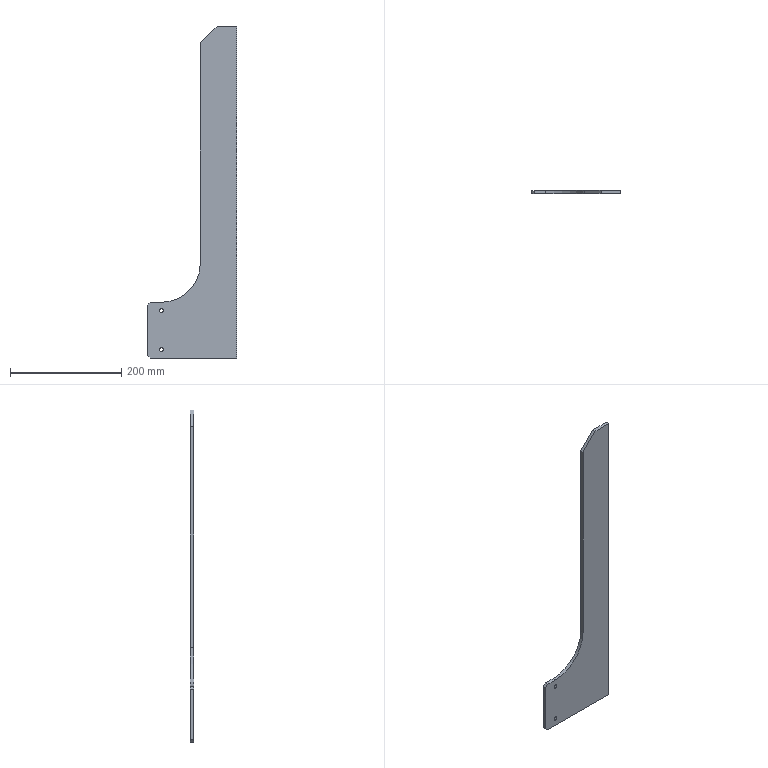Component | SolidWorks | THK-A1011BottomRibPlateLeft-2 | 1 solid | 16 faces | box 160 x 6 x 596 mm | volume 292463 mm3 | plane 11 | cylinder 5 | commonest cylinder face diameters 6.8 x4 140 x1 | material Q235A
build123d program:
from build123d import *

# Parameters (mm, degrees)
BOSS_EXTRUDE1_DEPTH = 3
CHAMFER1_SIZE       = 30
M8_TAPPED_HOLE1_D   = 6.8
CHAMFER2_SIZE       = 5


with BuildPart() as part:
    # Sketch1 → Boss-Extrude1 (new, symmetric)
    with BuildSketch(Plane(origin=(0, 0, 0), x_dir=(1, 0, 0), z_dir=(0, 1, 0))):
        with BuildLine():
            Line((0, 0), (0, -596))
            Line((0, -596), (-65, -596))
            Line((-65, -596), (-65, -170))
            ThreePointArc((-65, -170), (-85.503, -120.503), (-135, -100))
            Line((-135, -100), (-160, -100))
            Line((-160, -100), (-160, 0))
            Line((-160, 0), (0, 0))
        make_face()
    extrude(amount=BOSS_EXTRUDE1_DEPTH, both=True)

    # Chamfer1
    chamfer1_edges = [part.edges().sort_by_distance(p)[0] for p in [
        (-65, 0, 596),
    ]]
    chamfer(chamfer1_edges, length=CHAMFER1_SIZE)

    # M8 Tapped Hole1 (through all)
    with Locations(Plane(origin=(0, 3, 0), x_dir=(1, 0, 0), z_dir=(0, 1, 0))):
        with Locations((-135, -15), (-135, -85)):
            Hole(M8_TAPPED_HOLE1_D / 2)

    # Chamfer2
    chamfer2_edges = [part.edges().sort_by_distance(p)[0] for p in [
        (-160, 0, 100),
        (-160, 0, 0),
    ]]
    chamfer(chamfer2_edges, length=CHAMFER2_SIZE)


solid = part.part

# Placed as in the assembly
solid = solid.moved(Location((-73, -158, -371), (0, 0, 0)))
STEP:
#1=CARTESIAN_POINT('',(-8.189,-6.339,-14.15));
#2=VERTEX_POINT('',#1);
#3=CARTESIAN_POINT('',(-8.189,-6.339,-13.882));
#4=VERTEX_POINT('',#3);
#5=CARTESIAN_POINT('',(-8.189,-6.339,-14.016));
#6=DIRECTION('',(0.,1.,0.));
#7=DIRECTION('',(0.,0.,1.));
#8=AXIS2_PLACEMENT_3D('',#5,#6,#7);
#9=CIRCLE('',#8,0.1339);
#10=EDGE_CURVE('',#2,#4,#9,.T.);
#11=ORIENTED_EDGE('',*,*,#10,.F.);
#12=CARTESIAN_POINT('',(-8.189,-6.102,-14.15));
#13=VERTEX_POINT('',#12);
#14=CARTESIAN_POINT('',(-8.189,-6.102,-14.15));
#15=DIRECTION('',(0.,1.,0.));
#16=VECTOR('',#15,39.37);
#17=LINE('',#14,#16);
#18=EDGE_CURVE('',#2,#13,#17,.T.);
#19=ORIENTED_EDGE('',*,*,#18,.T.);
#20=CARTESIAN_POINT('',(-8.189,-6.102,-13.882));
#21=VERTEX_POINT('',#20);
#22=CARTESIAN_POINT('',(-8.189,-6.102,-14.016));
#23=DIRECTION('',(0.,1.,0.));
#24=DIRECTION('',(0.,0.,1.));
#25=AXIS2_PLACEMENT_3D('',#22,#23,#24);
#26=CIRCLE('',#25,0.1339);
#27=EDGE_CURVE('',#13,#21,#26,.T.);
#28=ORIENTED_EDGE('',*,*,#27,.T.);
#29=CARTESIAN_POINT('',(-8.189,-6.102,-13.882));
#30=DIRECTION('',(0.,1.,0.));
#31=VECTOR('',#30,39.37);
#32=LINE('',#29,#31);
#33=EDGE_CURVE('',#4,#21,#32,.T.);
#34=ORIENTED_EDGE('',*,*,#33,.F.);
#35=EDGE_LOOP('',(#11,#19,#28,#34));
#36=FACE_OUTER_BOUND('',#35,.T.);
#37=CARTESIAN_POINT('',(-8.189,-6.102,-14.016));
#38=DIRECTION('',(0.,1.,0.));
#39=DIRECTION('',(0.,0.,1.));
#40=AXIS2_PLACEMENT_3D('',#37,#38,#39);
#41=CYLINDRICAL_SURFACE('',#40,0.1339);
#42=ADVANCED_FACE('',(#36),#41,.F.);
#43=CARTESIAN_POINT('',(-8.189,-6.339,-11.394));
#44=VERTEX_POINT('',#43);
#45=CARTESIAN_POINT('',(-8.189,-6.339,-11.126));
#46=VERTEX_POINT('',#45);
#47=CARTESIAN_POINT('',(-8.189,-6.339,-11.26));
#48=DIRECTION('',(0.,1.,0.));
#49=DIRECTION('',(0.,0.,1.));
#50=AXIS2_PLACEMENT_3D('',#47,#48,#49);
#51=CIRCLE('',#50,0.1339);
#52=EDGE_CURVE('',#44,#46,#51,.T.);
#53=ORIENTED_EDGE('',*,*,#52,.F.);
#54=CARTESIAN_POINT('',(-8.189,-6.102,-11.394));
#55=VERTEX_POINT('',#54);
#56=CARTESIAN_POINT('',(-8.189,-6.102,-11.394));
#57=DIRECTION('',(0.,1.,0.));
#58=VECTOR('',#57,39.37);
#59=LINE('',#56,#58);
#60=EDGE_CURVE('',#44,#55,#59,.T.);
#61=ORIENTED_EDGE('',*,*,#60,.T.);
#62=CARTESIAN_POINT('',(-8.189,-6.102,-11.126));
#63=VERTEX_POINT('',#62);
#64=CARTESIAN_POINT('',(-8.189,-6.102,-11.26));
#65=DIRECTION('',(0.,1.,0.));
#66=DIRECTION('',(0.,0.,1.));
#67=AXIS2_PLACEMENT_3D('',#64,#65,#66);
#68=CIRCLE('',#67,0.1339);
#69=EDGE_CURVE('',#55,#63,#68,.T.);
#70=ORIENTED_EDGE('',*,*,#69,.T.);
#71=CARTESIAN_POINT('',(-8.189,-6.102,-11.126));
#72=DIRECTION('',(0.,1.,0.));
#73=VECTOR('',#72,39.37);
#74=LINE('',#71,#73);
#75=EDGE_CURVE('',#46,#63,#74,.T.);
#76=ORIENTED_EDGE('',*,*,#75,.F.);
#77=EDGE_LOOP('',(#53,#61,#70,#76));
#78=FACE_OUTER_BOUND('',#77,.T.);
#79=CARTESIAN_POINT('',(-8.189,-6.102,-11.26));
#80=DIRECTION('',(0.,1.,0.));
#81=DIRECTION('',(0.,0.,1.));
#82=AXIS2_PLACEMENT_3D('',#79,#80,#81);
#83=CYLINDRICAL_SURFACE('',#82,0.1339);
#84=ADVANCED_FACE('',(#78),#83,.F.);
#85=CARTESIAN_POINT('',(-2.874,-6.339,-14.606));
#86=VERTEX_POINT('',#85);
#87=CARTESIAN_POINT('',(-8.976,-6.339,-14.606));
#88=VERTEX_POINT('',#87);
#89=CARTESIAN_POINT('',(-2.874,-6.339,-14.606));
#90=DIRECTION('',(-1.,0.,0.));
#91=VECTOR('',#90,39.37);
#92=LINE('',#89,#91);
#93=EDGE_CURVE('',#86,#88,#92,.T.);
#94=ORIENTED_EDGE('',*,*,#93,.T.);
#95=CARTESIAN_POINT('',(-8.976,-6.102,-14.606));
#96=VERTEX_POINT('',#95);
#97=CARTESIAN_POINT('',(-8.976,-6.102,-14.606));
#98=DIRECTION('',(0.,1.,0.));
#99=VECTOR('',#98,39.37);
#100=LINE('',#97,#99);
#101=EDGE_CURVE('',#88,#96,#100,.T.);
#102=ORIENTED_EDGE('',*,*,#101,.T.);
#103=CARTESIAN_POINT('',(-2.874,-6.102,-14.606));
#104=VERTEX_POINT('',#103);
#105=CARTESIAN_POINT('',(-2.874,-6.102,-14.606));
#106=DIRECTION('',(-1.,0.,0.));
#107=VECTOR('',#106,39.37);
#108=LINE('',#105,#107);
#109=EDGE_CURVE('',#104,#96,#108,.T.);
#110=ORIENTED_EDGE('',*,*,#109,.F.);
#111=CARTESIAN_POINT('',(-2.874,-6.102,-14.606));
#112=DIRECTION('',(0.,-1.,0.));
#113=VECTOR('',#112,39.37);
#114=LINE('',#111,#113);
#115=EDGE_CURVE('',#104,#86,#114,.T.);
#116=ORIENTED_EDGE('',*,*,#115,.T.);
#117=EDGE_LOOP('',(#94,#102,#110,#116));
#118=FACE_OUTER_BOUND('',#117,.T.);
#119=CARTESIAN_POINT('',(-2.874,-6.102,-14.606));
#120=DIRECTION('',(0.,0.,1.));
#121=DIRECTION('',(1.,0.,-0.));
#122=AXIS2_PLACEMENT_3D('',#119,#120,#121);
#123=PLANE('',#122);
#124=ADVANCED_FACE('',(#118),#123,.F.);
#125=CARTESIAN_POINT('',(-9.173,-6.339,-14.409));
#126=VERTEX_POINT('',#125);
#127=CARTESIAN_POINT('',(-9.173,-6.339,-10.866));
#128=VERTEX_POINT('',#127);
#129=CARTESIAN_POINT('',(-9.173,-6.339,-14.606));
#130=DIRECTION('',(0.,0.,1.));
#131=VECTOR('',#130,39.37);
#132=LINE('',#129,#131);
#133=EDGE_CURVE('',#126,#128,#132,.T.);
#134=ORIENTED_EDGE('',*,*,#133,.T.);
#135=CARTESIAN_POINT('',(-9.173,-6.102,-10.866));
#136=VERTEX_POINT('',#135);
#137=CARTESIAN_POINT('',(-9.173,-6.102,-10.866));
#138=DIRECTION('',(0.,1.,0.));
#139=VECTOR('',#138,39.37);
#140=LINE('',#137,#139);
#141=EDGE_CURVE('',#128,#136,#140,.T.);
#142=ORIENTED_EDGE('',*,*,#141,.T.);
#143=CARTESIAN_POINT('',(-9.173,-6.102,-14.409));
#144=VERTEX_POINT('',#143);
#145=CARTESIAN_POINT('',(-9.173,-6.102,-14.606));
#146=DIRECTION('',(0.,0.,1.));
#147=VECTOR('',#146,39.37);
#148=LINE('',#145,#147);
#149=EDGE_CURVE('',#144,#136,#148,.T.);
#150=ORIENTED_EDGE('',*,*,#149,.F.);
#151=CARTESIAN_POINT('',(-9.173,-6.102,-14.409));
#152=DIRECTION('',(0.,-1.,0.));
#153=VECTOR('',#152,39.37);
#154=LINE('',#151,#153);
#155=EDGE_CURVE('',#144,#126,#154,.T.);
#156=ORIENTED_EDGE('',*,*,#155,.T.);
#157=EDGE_LOOP('',(#134,#142,#150,#156));
#158=FACE_OUTER_BOUND('',#157,.T.);
#159=CARTESIAN_POINT('',(-9.173,-6.102,-14.606));
#160=DIRECTION('',(1.,0.,0.));
#161=DIRECTION('',(0.,0.,-1.));
#162=AXIS2_PLACEMENT_3D('',#159,#160,#161);
#163=PLANE('',#162);
#164=ADVANCED_FACE('',(#158),#163,.F.);
#165=CARTESIAN_POINT('',(-8.976,-6.102,-10.669));
#166=VERTEX_POINT('',#165);
#167=CARTESIAN_POINT('',(-8.189,-6.102,-10.669));
#168=VERTEX_POINT('',#167);
#169=CARTESIAN_POINT('',(-8.189,-6.102,-10.669));
#170=DIRECTION('',(1.,0.,0.));
#171=VECTOR('',#170,39.37);
#172=LINE('',#169,#171);
#173=EDGE_CURVE('',#166,#168,#172,.T.);
#174=ORIENTED_EDGE('',*,*,#173,.F.);
#175=CARTESIAN_POINT('',(-8.976,-6.339,-10.669));
#176=VERTEX_POINT('',#175);
#177=CARTESIAN_POINT('',(-8.976,-6.102,-10.669));
#178=DIRECTION('',(0.,-1.,0.));
#179=VECTOR('',#178,39.37);
#180=LINE('',#177,#179);
#181=EDGE_CURVE('',#166,#176,#180,.T.);
#182=ORIENTED_EDGE('',*,*,#181,.T.);
#183=CARTESIAN_POINT('',(-8.189,-6.339,-10.669));
#184=VERTEX_POINT('',#183);
#185=CARTESIAN_POINT('',(-8.189,-6.339,-10.669));
#186=DIRECTION('',(1.,0.,0.));
#187=VECTOR('',#186,39.37);
#188=LINE('',#185,#187);
#189=EDGE_CURVE('',#176,#184,#188,.T.);
#190=ORIENTED_EDGE('',*,*,#189,.T.);
#191=CARTESIAN_POINT('',(-8.189,-6.102,-10.669));
#192=DIRECTION('',(0.,-1.,0.));
#193=VECTOR('',#192,39.37);
#194=LINE('',#191,#193);
#195=EDGE_CURVE('',#168,#184,#194,.T.);
#196=ORIENTED_EDGE('',*,*,#195,.F.);
#197=EDGE_LOOP('',(#174,#182,#190,#196));
#198=FACE_OUTER_BOUND('',#197,.T.);
#199=CARTESIAN_POINT('',(-8.189,-6.102,-10.669));
#200=DIRECTION('',(0.,0.,-1.));
#201=DIRECTION('',(-1.,0.,0.));
#202=AXIS2_PLACEMENT_3D('',#199,#200,#201);
#203=PLANE('',#202);
#204=ADVANCED_FACE('',(#198),#203,.F.);
#205=CARTESIAN_POINT('',(-5.433,-6.339,-7.913));
#206=VERTEX_POINT('',#205);
#207=CARTESIAN_POINT('',(-8.189,-6.339,-7.913));
#208=DIRECTION('',(0.,-1.,0.));
#209=DIRECTION('',(0.,0.,1.));
#210=AXIS2_PLACEMENT_3D('',#207,#208,#209);
#211=CIRCLE('',#210,2.756);
#212=EDGE_CURVE('',#184,#206,#211,.T.);
#213=ORIENTED_EDGE('',*,*,#212,.T.);
#214=CARTESIAN_POINT('',(-5.433,-6.102,-7.913));
#215=VERTEX_POINT('',#214);
#216=CARTESIAN_POINT('',(-5.433,-6.102,-7.913));
#217=DIRECTION('',(0.,-1.,0.));
#218=VECTOR('',#217,39.37);
#219=LINE('',#216,#218);
#220=EDGE_CURVE('',#215,#206,#219,.T.);
#221=ORIENTED_EDGE('',*,*,#220,.F.);
#222=CARTESIAN_POINT('',(-8.189,-6.102,-7.913));
#223=DIRECTION('',(0.,-1.,0.));
#224=DIRECTION('',(0.,0.,1.));
#225=AXIS2_PLACEMENT_3D('',#222,#223,#224);
#226=CIRCLE('',#225,2.756);
#227=EDGE_CURVE('',#168,#215,#226,.T.);
#228=ORIENTED_EDGE('',*,*,#227,.F.);
#229=ORIENTED_EDGE('',*,*,#195,.T.);
#230=EDGE_LOOP('',(#213,#221,#228,#229));
#231=FACE_OUTER_BOUND('',#230,.T.);
#232=CARTESIAN_POINT('',(-8.189,-6.102,-7.913));
#233=DIRECTION('',(0.,-1.,0.));
#234=DIRECTION('',(0.,0.,-1.));
#235=AXIS2_PLACEMENT_3D('',#232,#233,#234);
#236=CYLINDRICAL_SURFACE('',#235,2.756);
#237=ADVANCED_FACE('',(#231),#236,.F.);
#238=CARTESIAN_POINT('',(-5.433,-6.339,7.677));
#239=VERTEX_POINT('',#238);
#240=CARTESIAN_POINT('',(-5.433,-6.339,-7.913));
#241=DIRECTION('',(0.,0.,1.));
#242=VECTOR('',#241,39.37);
#243=LINE('',#240,#242);
#244=EDGE_CURVE('',#206,#239,#243,.T.);
#245=ORIENTED_EDGE('',*,*,#244,.T.);
#246=CARTESIAN_POINT('',(-5.433,-6.102,7.677));
#247=VERTEX_POINT('',#246);
#248=CARTESIAN_POINT('',(-5.433,-6.102,7.677));
#249=DIRECTION('',(0.,1.,0.));
#250=VECTOR('',#249,39.37);
#251=LINE('',#248,#250);
#252=EDGE_CURVE('',#239,#247,#251,.T.);
#253=ORIENTED_EDGE('',*,*,#252,.T.);
#254=CARTESIAN_POINT('',(-5.433,-6.102,-7.913));
#255=DIRECTION('',(0.,0.,1.));
#256=VECTOR('',#255,39.37);
#257=LINE('',#254,#256);
#258=EDGE_CURVE('',#215,#247,#257,.T.);
#259=ORIENTED_EDGE('',*,*,#258,.F.);
#260=ORIENTED_EDGE('',*,*,#220,.T.);
#261=EDGE_LOOP('',(#245,#253,#259,#260));
#262=FACE_OUTER_BOUND('',#261,.T.);
#263=CARTESIAN_POINT('',(-5.433,-6.102,-7.913));
#264=DIRECTION('',(1.,0.,-0.));
#265=DIRECTION('',(-0.,0.,-1.));
#266=AXIS2_PLACEMENT_3D('',#263,#264,#265);
#267=PLANE('',#266);
#268=ADVANCED_FACE('',(#262),#267,.F.);
#269=CARTESIAN_POINT('',(-4.252,-6.102,8.858));
#270=VERTEX_POINT('',#269);
#271=CARTESIAN_POINT('',(-2.874,-6.102,8.858));
#272=VERTEX_POINT('',#271);
#273=CARTESIAN_POINT('',(-5.433,-6.102,8.858));
#274=DIRECTION('',(1.,0.,0.));
#275=VECTOR('',#274,39.37);
#276=LINE('',#273,#275);
#277=EDGE_CURVE('',#270,#272,#276,.T.);
#278=ORIENTED_EDGE('',*,*,#277,.F.);
#279=CARTESIAN_POINT('',(-4.252,-6.339,8.858));
#280=VERTEX_POINT('',#279);
#281=CARTESIAN_POINT('',(-4.252,-6.102,8.858));
#282=DIRECTION('',(0.,-1.,0.));
#283=VECTOR('',#282,39.37);
#284=LINE('',#281,#283);
#285=EDGE_CURVE('',#270,#280,#284,.T.);
#286=ORIENTED_EDGE('',*,*,#285,.T.);
#287=CARTESIAN_POINT('',(-2.874,-6.339,8.858));
#288=VERTEX_POINT('',#287);
#289=CARTESIAN_POINT('',(-5.433,-6.339,8.858));
#290=DIRECTION('',(1.,0.,0.));
#291=VECTOR('',#290,39.37);
#292=LINE('',#289,#291);
#293=EDGE_CURVE('',#280,#288,#292,.T.);
#294=ORIENTED_EDGE('',*,*,#293,.T.);
#295=CARTESIAN_POINT('',(-2.874,-6.102,8.858));
#296=DIRECTION('',(0.,-1.,0.));
#297=VECTOR('',#296,39.37);
#298=LINE('',#295,#297);
#299=EDGE_CURVE('',#272,#288,#298,.T.);
#300=ORIENTED_EDGE('',*,*,#299,.F.);
#301=EDGE_LOOP('',(#278,#286,#294,#300));
#302=FACE_OUTER_BOUND('',#301,.T.);
#303=CARTESIAN_POINT('',(-5.433,-6.102,8.858));
#304=DIRECTION('',(0.,0.,-1.));
#305=DIRECTION('',(-1.,0.,0.));
#306=AXIS2_PLACEMENT_3D('',#303,#304,#305);
#307=PLANE('',#306);
#308=ADVANCED_FACE('',(#302),#307,.F.);
#309=CARTESIAN_POINT('',(-2.874,-6.339,-14.606));
#310=DIRECTION('',(-0.,0.,-1.));
#311=VECTOR('',#310,39.37);
#312=LINE('',#309,#311);
#313=EDGE_CURVE('',#288,#86,#312,.T.);
#314=ORIENTED_EDGE('',*,*,#313,.T.);
#315=ORIENTED_EDGE('',*,*,#115,.F.);
#316=CARTESIAN_POINT('',(-2.874,-6.102,-14.606));
#317=DIRECTION('',(-0.,0.,-1.));
#318=VECTOR('',#317,39.37);
#319=LINE('',#316,#318);
#320=EDGE_CURVE('',#272,#104,#319,.T.);
#321=ORIENTED_EDGE('',*,*,#320,.F.);
#322=ORIENTED_EDGE('',*,*,#299,.T.);
#323=EDGE_LOOP('',(#314,#315,#321,#322));
#324=FACE_OUTER_BOUND('',#323,.T.);
#325=CARTESIAN_POINT('',(-2.874,-6.102,-14.606));
#326=DIRECTION('',(-1.,0.,0.));
#327=DIRECTION('',(0.,0.,1.));
#328=AXIS2_PLACEMENT_3D('',#325,#326,#327);
#329=PLANE('',#328);
#330=ADVANCED_FACE('',(#324),#329,.F.);
#331=CARTESIAN_POINT('',(-8.189,-6.102,-14.016));
#332=DIRECTION('',(0.,1.,0.));
#333=DIRECTION('',(0.,0.,1.));
#334=AXIS2_PLACEMENT_3D('',#331,#332,#333);
#335=CIRCLE('',#334,0.1339);
#336=EDGE_CURVE('',#21,#13,#335,.T.);
#337=ORIENTED_EDGE('',*,*,#336,.F.);
#338=ORIENTED_EDGE('',*,*,#27,.F.);
#339=EDGE_LOOP('',(#337,#338));
#340=FACE_BOUND('',#339,.T.);
#341=CARTESIAN_POINT('',(-8.189,-6.102,-11.26));
#342=DIRECTION('',(0.,1.,0.));
#343=DIRECTION('',(0.,0.,1.));
#344=AXIS2_PLACEMENT_3D('',#341,#342,#343);
#345=CIRCLE('',#344,0.1339);
#346=EDGE_CURVE('',#63,#55,#345,.T.);
#347=ORIENTED_EDGE('',*,*,#346,.F.);
#348=ORIENTED_EDGE('',*,*,#69,.F.);
#349=EDGE_LOOP('',(#347,#348));
#350=FACE_BOUND('',#349,.T.);
#351=ORIENTED_EDGE('',*,*,#149,.T.);
#352=CARTESIAN_POINT('',(-7.205,-6.102,-8.898));
#353=DIRECTION('',(0.7071,0.,0.7071));
#354=VECTOR('',#353,39.37);
#355=LINE('',#352,#354);
#356=EDGE_CURVE('',#136,#166,#355,.T.);
#357=ORIENTED_EDGE('',*,*,#356,.T.);
#358=ORIENTED_EDGE('',*,*,#173,.T.);
#359=ORIENTED_EDGE('',*,*,#227,.T.);
#360=ORIENTED_EDGE('',*,*,#258,.T.);
#361=CARTESIAN_POINT('',(-14.606,-6.102,-1.496));
#362=DIRECTION('',(0.7071,0.,0.7071));
#363=VECTOR('',#362,39.37);
#364=LINE('',#361,#363);
#365=EDGE_CURVE('',#247,#270,#364,.T.);
#366=ORIENTED_EDGE('',*,*,#365,.T.);
#367=ORIENTED_EDGE('',*,*,#277,.T.);
#368=ORIENTED_EDGE('',*,*,#320,.T.);
#369=ORIENTED_EDGE('',*,*,#109,.T.);
#370=CARTESIAN_POINT('',(-11.929,-6.102,-11.654));
#371=DIRECTION('',(-0.7071,0.,0.7071));
#372=VECTOR('',#371,39.37);
#373=LINE('',#370,#372);
#374=EDGE_CURVE('',#96,#144,#373,.T.);
#375=ORIENTED_EDGE('',*,*,#374,.T.);
#376=EDGE_LOOP('',(#351,#357,#358,#359,#360,#366,#367,#368,#369,#375));
#377=FACE_OUTER_BOUND('',#376,.T.);
#378=CARTESIAN_POINT('',(-8.189,-6.102,-7.913));
#379=DIRECTION('',(0.,1.,0.));
#380=DIRECTION('',(0.,0.,1.));
#381=AXIS2_PLACEMENT_3D('',#378,#379,#380);
#382=PLANE('',#381);
#383=ADVANCED_FACE('',(#340,#350,#377),#382,.T.);
#384=CARTESIAN_POINT('',(-8.189,-6.339,-14.016));
#385=DIRECTION('',(0.,1.,0.));
#386=DIRECTION('',(0.,0.,1.));
#387=AXIS2_PLACEMENT_3D('',#384,#385,#386);
#388=CIRCLE('',#387,0.1339);
#389=EDGE_CURVE('',#4,#2,#388,.T.);
#390=ORIENTED_EDGE('',*,*,#389,.T.);
#391=ORIENTED_EDGE('',*,*,#10,.T.);
#392=EDGE_LOOP('',(#390,#391));
#393=FACE_BOUND('',#392,.T.);
#394=CARTESIAN_POINT('',(-8.189,-6.339,-11.26));
#395=DIRECTION('',(0.,1.,0.));
#396=DIRECTION('',(0.,0.,1.));
#397=AXIS2_PLACEMENT_3D('',#394,#395,#396);
#398=CIRCLE('',#397,0.1339);
#399=EDGE_CURVE('',#46,#44,#398,.T.);
#400=ORIENTED_EDGE('',*,*,#399,.T.);
#401=ORIENTED_EDGE('',*,*,#52,.T.);
#402=EDGE_LOOP('',(#400,#401));
#403=FACE_BOUND('',#402,.T.);
#404=ORIENTED_EDGE('',*,*,#189,.F.);
#405=CARTESIAN_POINT('',(-8.976,-6.339,-10.669));
#406=DIRECTION('',(-0.7071,0.,-0.7071));
#407=VECTOR('',#406,39.37);
#408=LINE('',#405,#407);
#409=EDGE_CURVE('',#176,#128,#408,.T.);
#410=ORIENTED_EDGE('',*,*,#409,.T.);
#411=ORIENTED_EDGE('',*,*,#133,.F.);
#412=CARTESIAN_POINT('',(-9.173,-6.339,-14.409));
#413=DIRECTION('',(0.7071,0.,-0.7071));
#414=VECTOR('',#413,39.37);
#415=LINE('',#412,#414);
#416=EDGE_CURVE('',#126,#88,#415,.T.);
#417=ORIENTED_EDGE('',*,*,#416,.T.);
#418=ORIENTED_EDGE('',*,*,#93,.F.);
#419=ORIENTED_EDGE('',*,*,#313,.F.);
#420=ORIENTED_EDGE('',*,*,#293,.F.);
#421=CARTESIAN_POINT('',(-4.252,-6.339,8.858));
#422=DIRECTION('',(-0.7071,0.,-0.7071));
#423=VECTOR('',#422,39.37);
#424=LINE('',#421,#423);
#425=EDGE_CURVE('',#280,#239,#424,.T.);
#426=ORIENTED_EDGE('',*,*,#425,.T.);
#427=ORIENTED_EDGE('',*,*,#244,.F.);
#428=ORIENTED_EDGE('',*,*,#212,.F.);
#429=EDGE_LOOP('',(#404,#410,#411,#417,#418,#419,#420,#426,#427,#428));
#430=FACE_OUTER_BOUND('',#429,.T.);
#431=CARTESIAN_POINT('',(-8.189,-6.339,-7.913));
#432=DIRECTION('',(0.,1.,0.));
#433=DIRECTION('',(0.,0.,1.));
#434=AXIS2_PLACEMENT_3D('',#431,#432,#433);
#435=PLANE('',#434);
#436=ADVANCED_FACE('',(#393,#403,#430),#435,.F.);
#437=ORIENTED_EDGE('',*,*,#365,.F.);
#438=ORIENTED_EDGE('',*,*,#252,.F.);
#439=ORIENTED_EDGE('',*,*,#425,.F.);
#440=ORIENTED_EDGE('',*,*,#285,.F.);
#441=EDGE_LOOP('',(#437,#438,#439,#440));
#442=FACE_OUTER_BOUND('',#441,.T.);
#443=CARTESIAN_POINT('',(-4.252,-6.102,8.858));
#444=DIRECTION('',(0.7071,0.,-0.7071));
#445=DIRECTION('',(0.,-1.,0.));
#446=AXIS2_PLACEMENT_3D('',#443,#444,#445);
#447=PLANE('',#446);
#448=ADVANCED_FACE('',(#442),#447,.F.);
#449=ORIENTED_EDGE('',*,*,#60,.F.);
#450=ORIENTED_EDGE('',*,*,#399,.F.);
#451=ORIENTED_EDGE('',*,*,#75,.T.);
#452=ORIENTED_EDGE('',*,*,#346,.T.);
#453=EDGE_LOOP('',(#449,#450,#451,#452));
#454=FACE_OUTER_BOUND('',#453,.T.);
#455=CARTESIAN_POINT('',(-8.189,-6.102,-11.26));
#456=DIRECTION('',(0.,1.,0.));
#457=DIRECTION('',(0.,0.,1.));
#458=AXIS2_PLACEMENT_3D('',#455,#456,#457);
#459=CYLINDRICAL_SURFACE('',#458,0.1339);
#460=ADVANCED_FACE('',(#454),#459,.F.);
#461=ORIENTED_EDGE('',*,*,#18,.F.);
#462=ORIENTED_EDGE('',*,*,#389,.F.);
#463=ORIENTED_EDGE('',*,*,#33,.T.);
#464=ORIENTED_EDGE('',*,*,#336,.T.);
#465=EDGE_LOOP('',(#461,#462,#463,#464));
#466=FACE_OUTER_BOUND('',#465,.T.);
#467=CARTESIAN_POINT('',(-8.189,-6.102,-14.016));
#468=DIRECTION('',(0.,1.,0.));
#469=DIRECTION('',(0.,0.,1.));
#470=AXIS2_PLACEMENT_3D('',#467,#468,#469);
#471=CYLINDRICAL_SURFACE('',#470,0.1339);
#472=ADVANCED_FACE('',(#466),#471,.F.);
#473=ORIENTED_EDGE('',*,*,#356,.F.);
#474=ORIENTED_EDGE('',*,*,#141,.F.);
#475=ORIENTED_EDGE('',*,*,#409,.F.);
#476=ORIENTED_EDGE('',*,*,#181,.F.);
#477=EDGE_LOOP('',(#473,#474,#475,#476));
#478=FACE_OUTER_BOUND('',#477,.T.);
#479=CARTESIAN_POINT('',(-8.976,-6.102,-10.669));
#480=DIRECTION('',(0.7071,0.,-0.7071));
#481=DIRECTION('',(0.,-1.,0.));
#482=AXIS2_PLACEMENT_3D('',#479,#480,#481);
#483=PLANE('',#482);
#484=ADVANCED_FACE('',(#478),#483,.F.);
#485=ORIENTED_EDGE('',*,*,#374,.F.);
#486=ORIENTED_EDGE('',*,*,#101,.F.);
#487=ORIENTED_EDGE('',*,*,#416,.F.);
#488=ORIENTED_EDGE('',*,*,#155,.F.);
#489=EDGE_LOOP('',(#485,#486,#487,#488));
#490=FACE_OUTER_BOUND('',#489,.T.);
#491=CARTESIAN_POINT('',(-9.173,-6.102,-14.409));
#492=DIRECTION('',(0.7071,0.,0.7071));
#493=DIRECTION('',(0.,-1.,0.));
#494=AXIS2_PLACEMENT_3D('',#491,#492,#493);
#495=PLANE('',#494);
#496=ADVANCED_FACE('',(#490),#495,.F.);
#497=CLOSED_SHELL('',(#42,#84,#124,#164,#204,#237,#268,#308,#330,#383,#436,#448,#460,#472,#484,#496));
#498=MANIFOLD_SOLID_BREP('',#497);
#499=CARTESIAN_POINT('',(0.,0.,0.));
#500=DIRECTION('',(0.,0.,1.));
#501=DIRECTION('',(1.,0.,0.));
#502=AXIS2_PLACEMENT_3D('',#499,#500,#501);
#503=(LENGTH_UNIT()NAMED_UNIT(*)SI_UNIT($,.METRE.));
#504=LENGTH_MEASURE_WITH_UNIT(LENGTH_MEASURE(0.0254),#503);
#505=DIMENSIONAL_EXPONENTS(1.,0.,0.,0.,0.,0.,0.);
#506=(CONVERSION_BASED_UNIT('',#504)LENGTH_UNIT()NAMED_UNIT(#505));
#507=UNCERTAINTY_MEASURE_WITH_UNIT(LENGTH_MEASURE(0.00001),#506,'','');
#508=(NAMED_UNIT(*)PLANE_ANGLE_UNIT()SI_UNIT($,.RADIAN.));
#509=(NAMED_UNIT(*)SI_UNIT($,.STERADIAN.)SOLID_ANGLE_UNIT());
#510=(GEOMETRIC_REPRESENTATION_CONTEXT(3)GLOBAL_UNCERTAINTY_ASSIGNED_CONTEXT((#507))GLOBAL_UNIT_ASSIGNED_CONTEXT((#506,#508,#509))REPRESENTATION_CONTEXT('',''));
#511=ADVANCED_BREP_SHAPE_REPRESENTATION('',(#498,#502),#510);
#512=COLOUR_RGB('',0.7922,0.8196,0.9333);
#513=FILL_AREA_STYLE_COLOUR('',#512);
#514=FILL_AREA_STYLE('',(#513));
#515=SURFACE_STYLE_FILL_AREA(#514);
#516=SURFACE_SIDE_STYLE('',(#515));
#517=SURFACE_STYLE_USAGE(.BOTH.,#516);
#518=PRESENTATION_STYLE_ASSIGNMENT((#517));
#519=STYLED_ITEM('',(#518),#498);
#520=PRESENTATION_LAYER_ASSIGNMENT('','',(#519));
#521=(LENGTH_UNIT()NAMED_UNIT(*)SI_UNIT($,.METRE.));
#522=LENGTH_MEASURE_WITH_UNIT(LENGTH_MEASURE(0.0254),#521);
#523=DIMENSIONAL_EXPONENTS(1.,0.,0.,0.,0.,0.,0.);
#524=(CONVERSION_BASED_UNIT('',#522)LENGTH_UNIT()NAMED_UNIT(#523));
#525=UNCERTAINTY_MEASURE_WITH_UNIT(LENGTH_MEASURE(0.00001),#524,'','');
#526=(NAMED_UNIT(*)PLANE_ANGLE_UNIT()SI_UNIT($,.RADIAN.));
#527=(NAMED_UNIT(*)SI_UNIT($,.STERADIAN.)SOLID_ANGLE_UNIT());
#528=(GEOMETRIC_REPRESENTATION_CONTEXT(3)GLOBAL_UNCERTAINTY_ASSIGNED_CONTEXT((#525))GLOBAL_UNIT_ASSIGNED_CONTEXT((#524,#526,#527))REPRESENTATION_CONTEXT('',''));
#529=MECHANICAL_DESIGN_GEOMETRIC_PRESENTATION_REPRESENTATION('',(#519),#528);